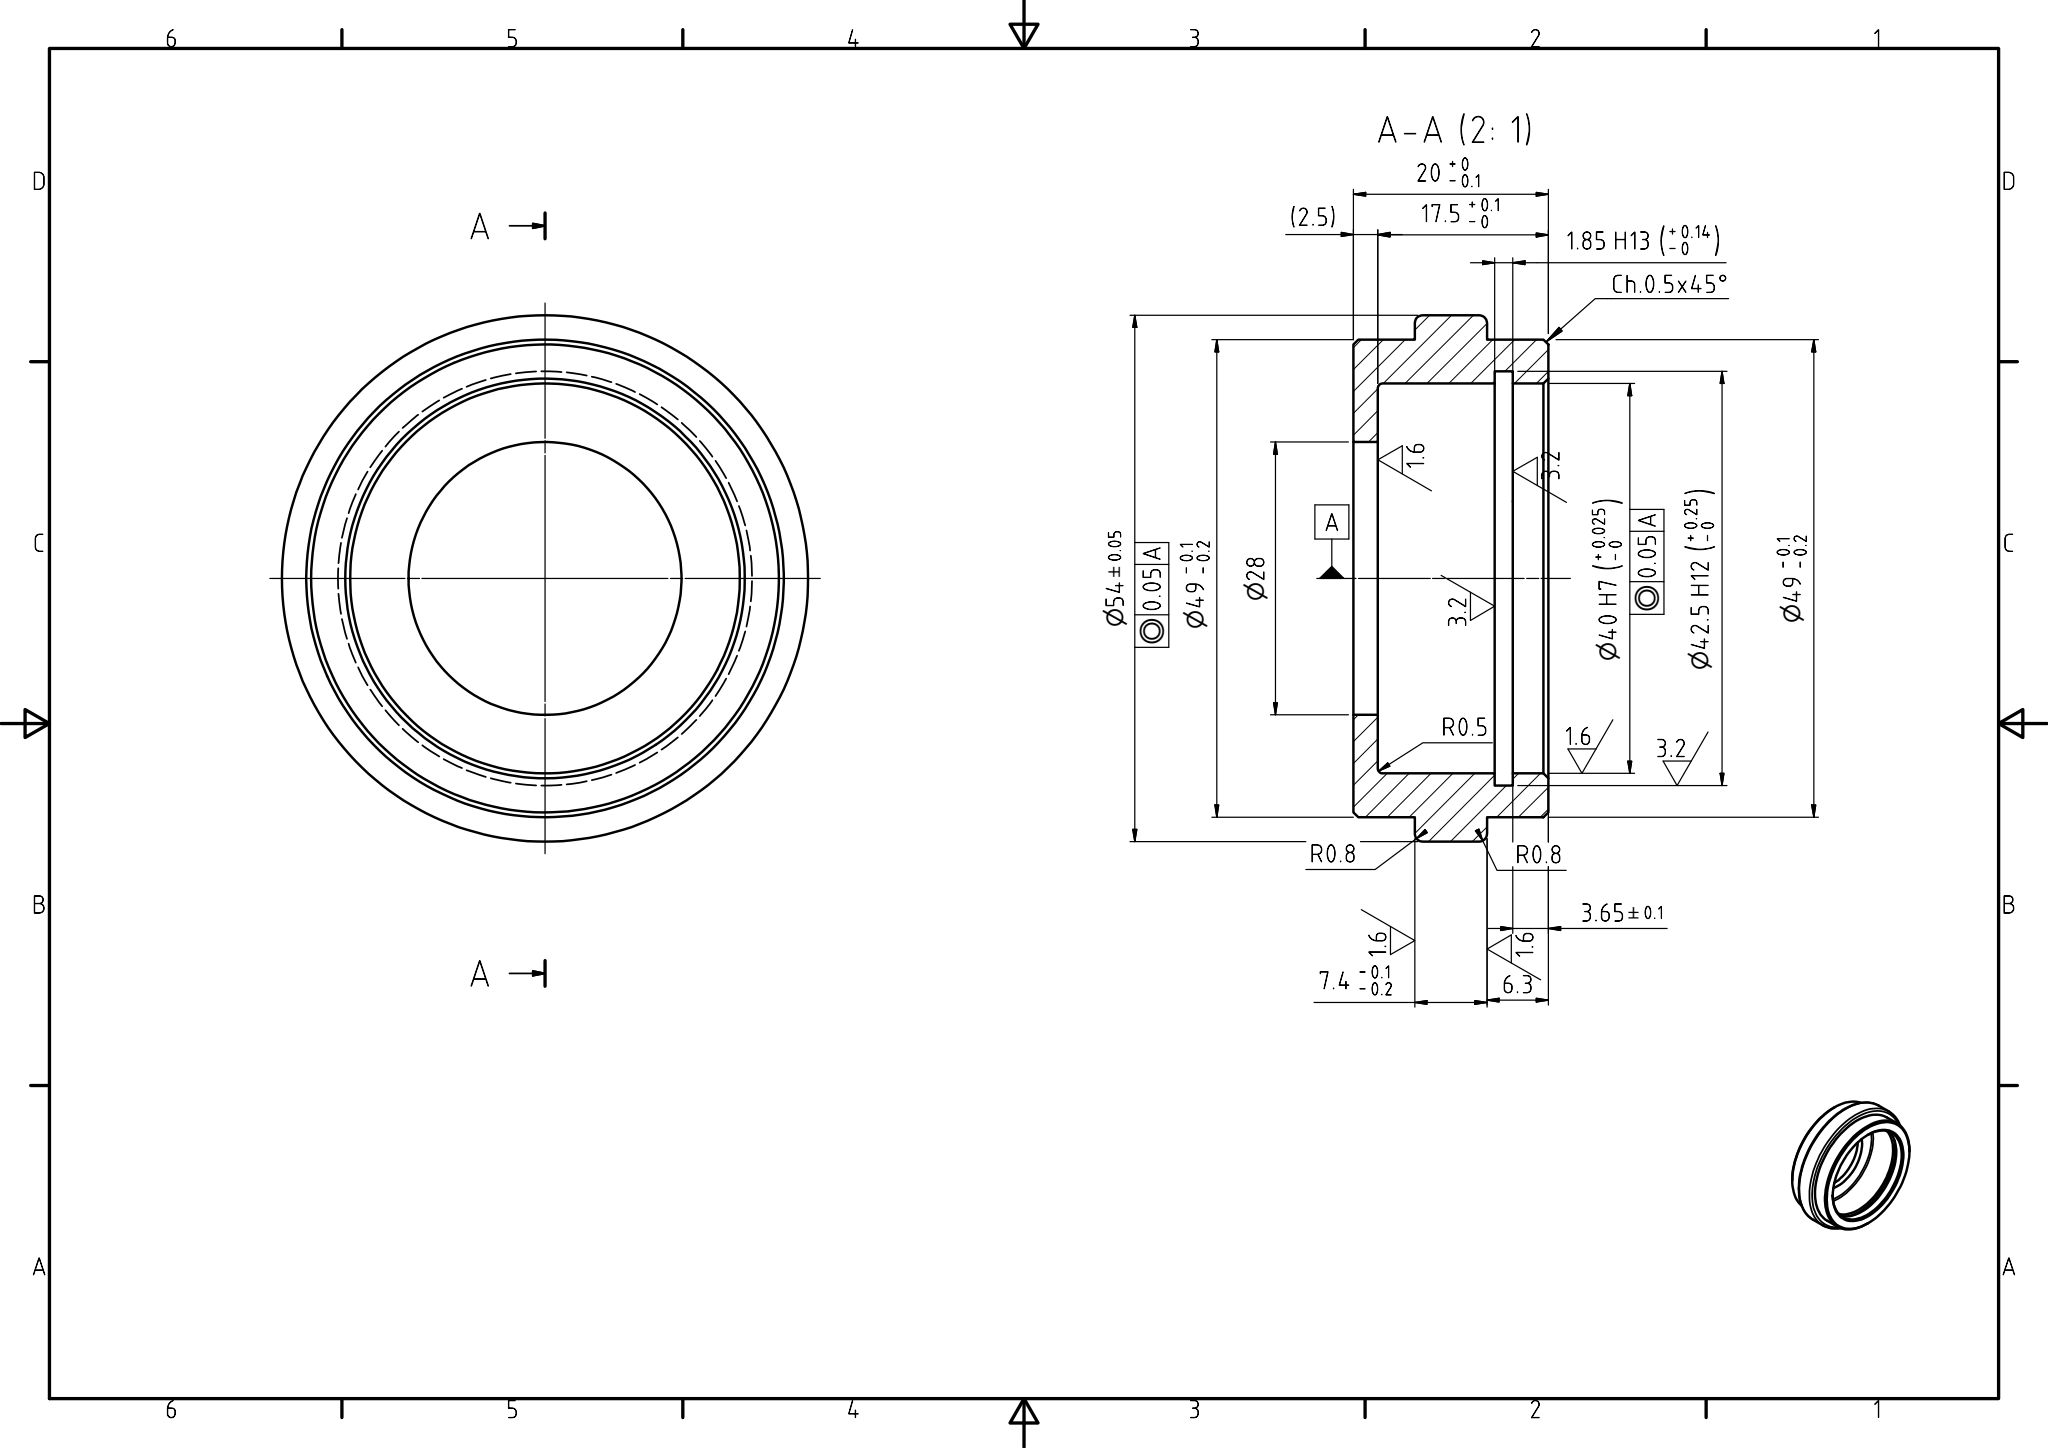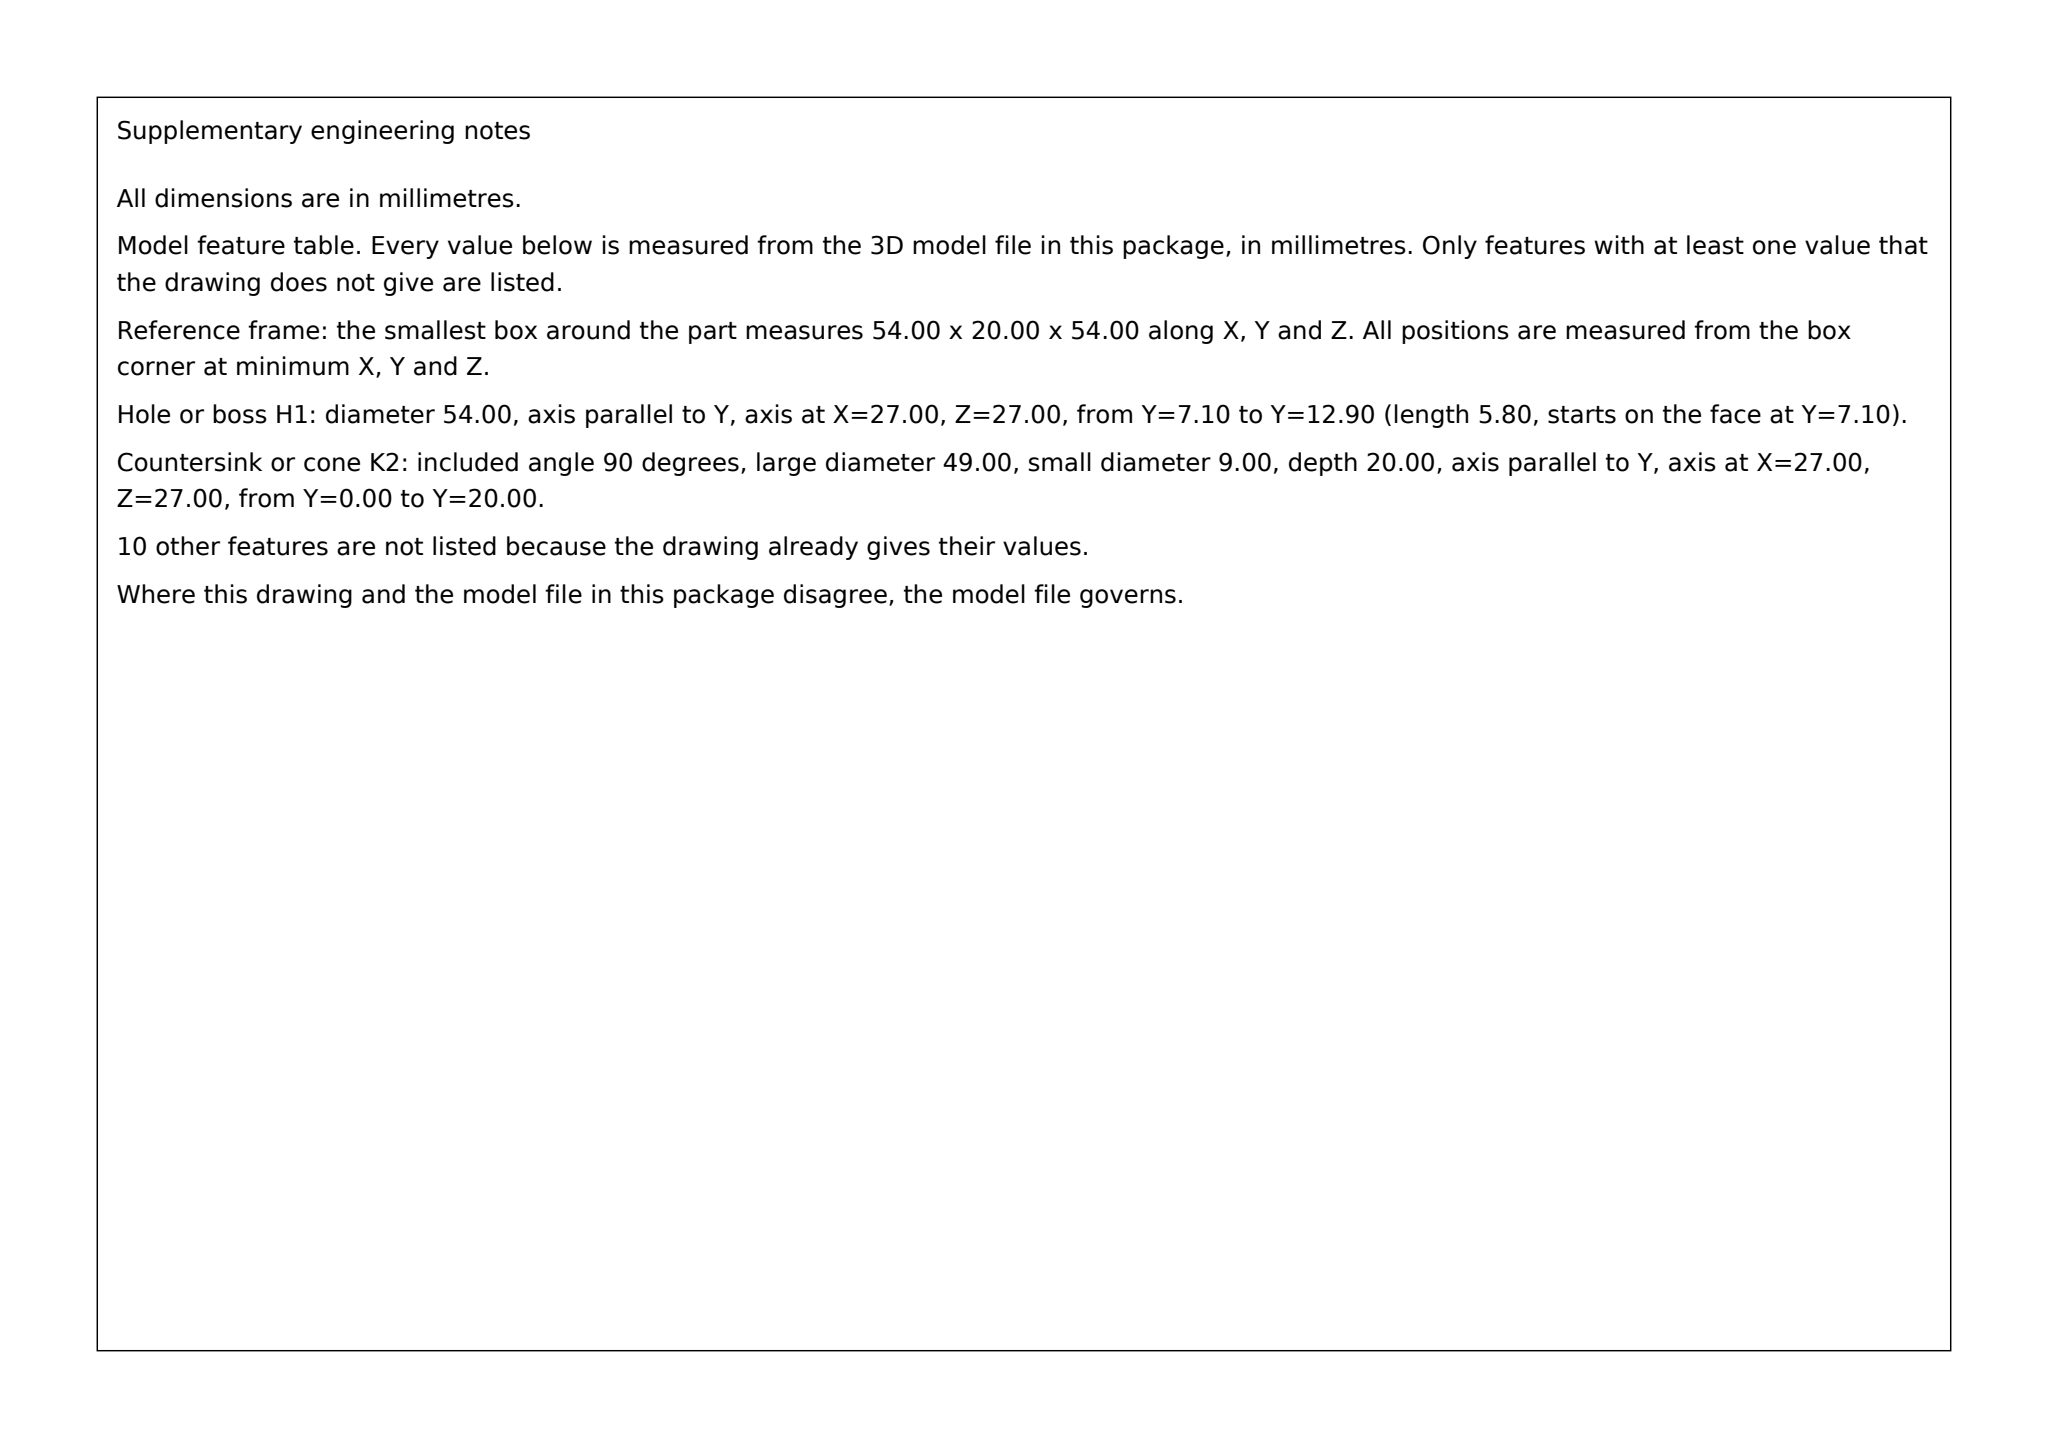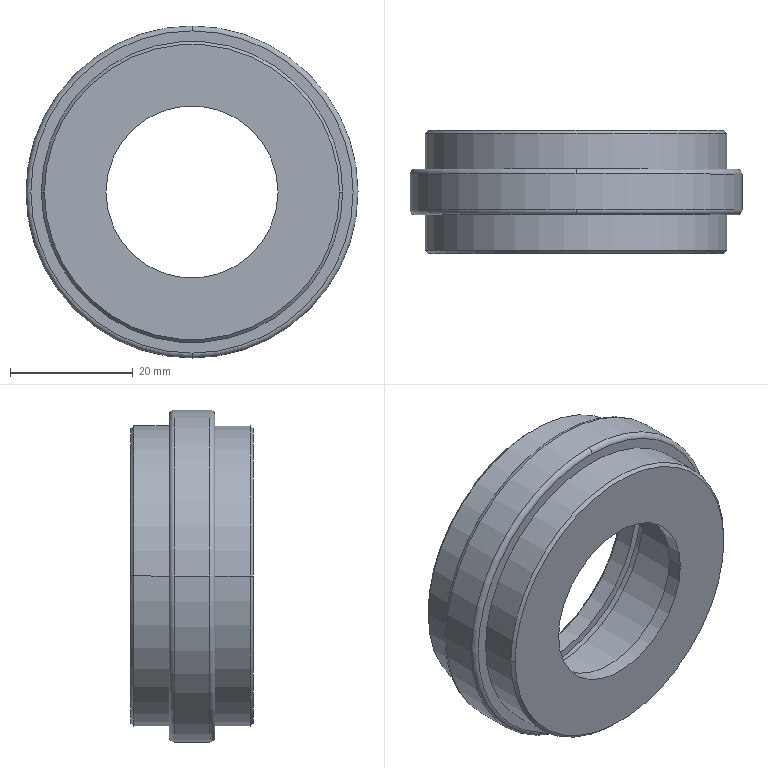Part | SolidWorks | mm | 1 solid | 33 faces | box 54 x 20 x 54 mm | volume 16784 mm3 | cylinder 14 | plane 7 | cone 6 | torus 6 | commonest cylinder face diameters 40 x4 49 x4 28 x2 42.5 x2 54 x2